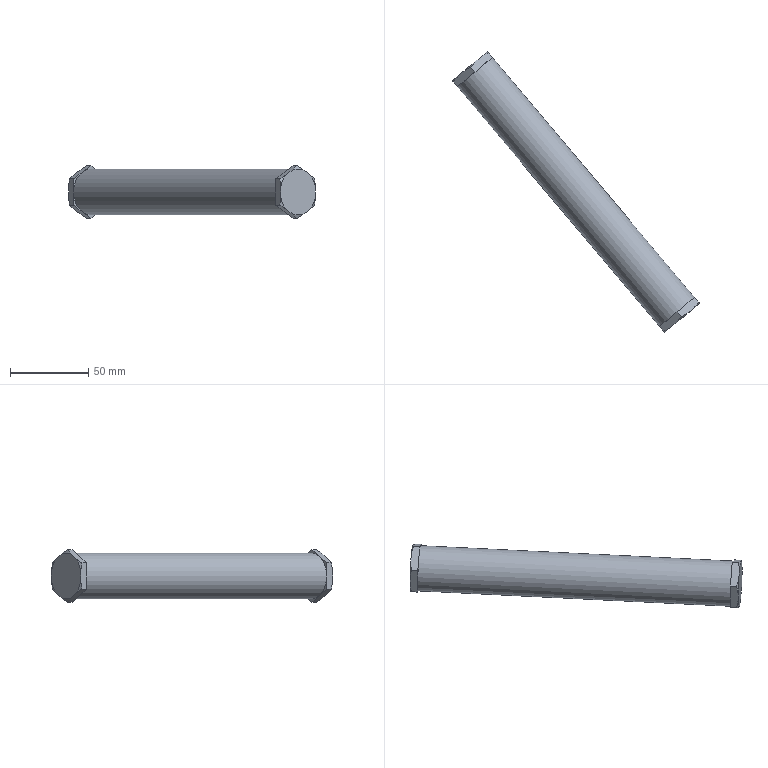Component | NX | PERNO3 | 1 solid | 39 faces | volume 139356 mm3 | plane 26 | cone 12 | cylinder 1 | commonest cylinder face diameters 29 x1